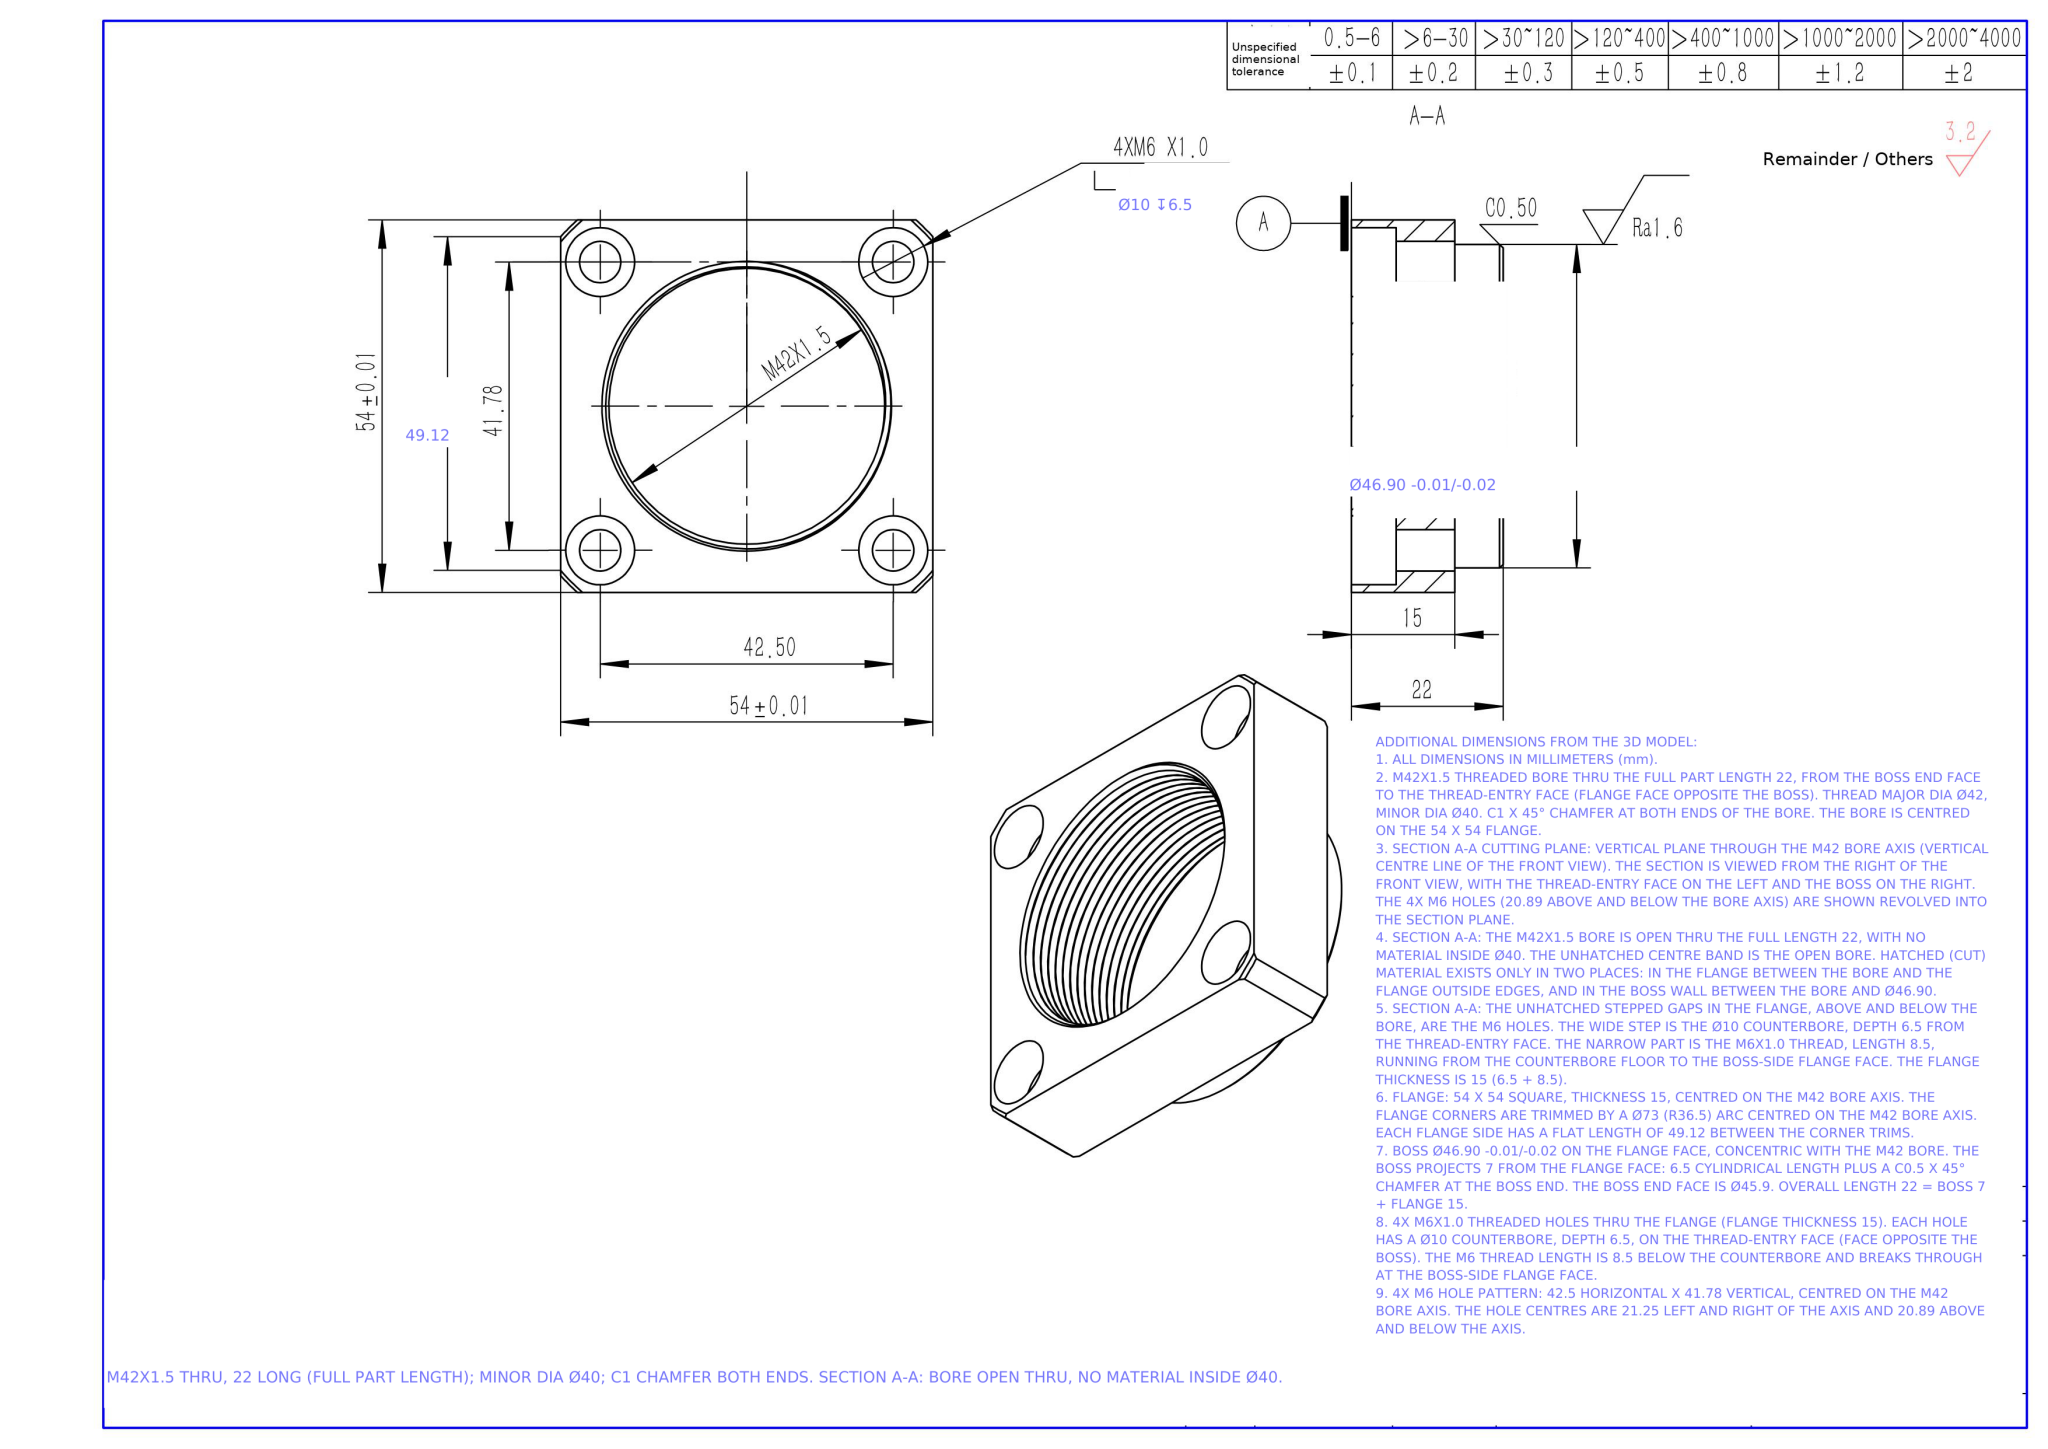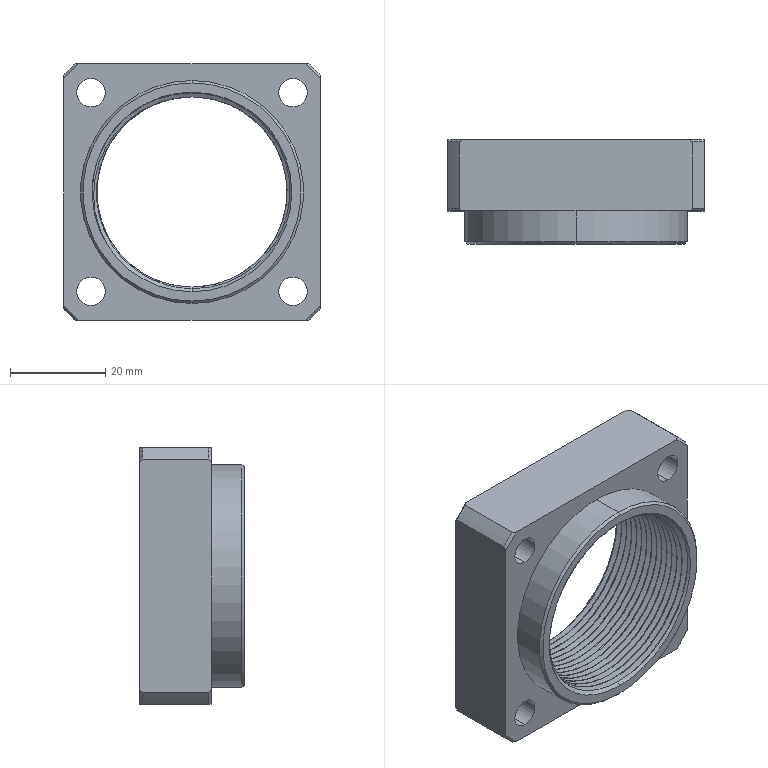Part | NX | mm | 1 solid | 110 faces | box 54 x 22 x 54 mm | volume 23390 mm3 | cylinder 80 | cone 17 | plane 11 | spline 2 | commonest cylinder face diameters 42 x30 40 x28 10 x8 6 x8 73 x4 46.9 x2